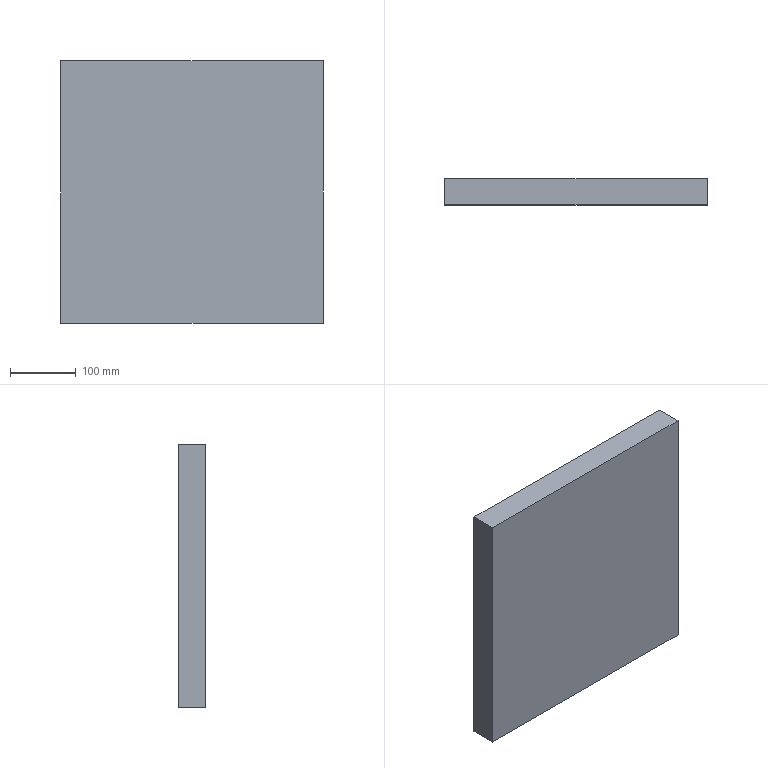Component | SolidWorks | DieBasePlate-1 | 1 solid | 6 faces | box 400 x 40 x 400 mm | volume 6400000 mm3 | plane 6
build123d program:
from build123d import *

# Parameters (mm, degrees)
SKETCH1_W           = 400
SKETCH1_H           = 400
BOSS_EXTRUDE1_DEPTH = 40


with BuildPart() as part:
    # Sketch1 → Boss-Extrude1 (new body)
    with BuildSketch(Plane.XY):
        with Locations((200, 200)):
            Rectangle(SKETCH1_W, SKETCH1_H)
    extrude(amount=BOSS_EXTRUDE1_DEPTH)


solid = part.part

# Placed as in the assembly
solid = solid.moved(Location((-377.951, 437.323, -195), (90, 0, 0)))
STEP:
#1=CARTESIAN_POINT('',(-14.88,15.643,-7.677));
#2=VERTEX_POINT('',#1);
#3=CARTESIAN_POINT('',(-14.88,15.643,8.071));
#4=VERTEX_POINT('',#3);
#5=CARTESIAN_POINT('',(-14.88,15.643,8.071));
#6=DIRECTION('',(0.,-0.,1.));
#7=VECTOR('',#6,39.37);
#8=LINE('',#5,#7);
#9=EDGE_CURVE('',#2,#4,#8,.T.);
#10=ORIENTED_EDGE('',*,*,#9,.T.);
#11=CARTESIAN_POINT('',(-14.88,17.217,8.071));
#12=VERTEX_POINT('',#11);
#13=CARTESIAN_POINT('',(-14.88,17.217,8.071));
#14=DIRECTION('',(-0.,-1.,-0.));
#15=VECTOR('',#14,39.37);
#16=LINE('',#13,#15);
#17=EDGE_CURVE('',#12,#4,#16,.T.);
#18=ORIENTED_EDGE('',*,*,#17,.F.);
#19=CARTESIAN_POINT('',(-14.88,17.217,-7.677));
#20=VERTEX_POINT('',#19);
#21=CARTESIAN_POINT('',(-14.88,17.217,8.071));
#22=DIRECTION('',(0.,-0.,1.));
#23=VECTOR('',#22,39.37);
#24=LINE('',#21,#23);
#25=EDGE_CURVE('',#20,#12,#24,.T.);
#26=ORIENTED_EDGE('',*,*,#25,.F.);
#27=CARTESIAN_POINT('',(-14.88,17.217,-7.677));
#28=DIRECTION('',(-0.,-1.,-0.));
#29=VECTOR('',#28,39.37);
#30=LINE('',#27,#29);
#31=EDGE_CURVE('',#20,#2,#30,.T.);
#32=ORIENTED_EDGE('',*,*,#31,.T.);
#33=EDGE_LOOP('',(#10,#18,#26,#32));
#34=FACE_OUTER_BOUND('',#33,.T.);
#35=CARTESIAN_POINT('',(-14.88,17.217,8.071));
#36=DIRECTION('',(1.,-0.,-0.));
#37=DIRECTION('',(-0.,-1.,-0.));
#38=AXIS2_PLACEMENT_3D('',#35,#36,#37);
#39=PLANE('',#38);
#40=ADVANCED_FACE('',(#34),#39,.F.);
#41=CARTESIAN_POINT('',(0.8681,15.643,8.071));
#42=VERTEX_POINT('',#41);
#43=CARTESIAN_POINT('',(-14.88,15.643,8.071));
#44=DIRECTION('',(1.,-0.,-0.));
#45=VECTOR('',#44,39.37);
#46=LINE('',#43,#45);
#47=EDGE_CURVE('',#4,#42,#46,.T.);
#48=ORIENTED_EDGE('',*,*,#47,.T.);
#49=CARTESIAN_POINT('',(0.8681,17.217,8.071));
#50=VERTEX_POINT('',#49);
#51=CARTESIAN_POINT('',(0.8681,17.217,8.071));
#52=DIRECTION('',(-0.,-1.,-0.));
#53=VECTOR('',#52,39.37);
#54=LINE('',#51,#53);
#55=EDGE_CURVE('',#50,#42,#54,.T.);
#56=ORIENTED_EDGE('',*,*,#55,.F.);
#57=CARTESIAN_POINT('',(-14.88,17.217,8.071));
#58=DIRECTION('',(1.,-0.,-0.));
#59=VECTOR('',#58,39.37);
#60=LINE('',#57,#59);
#61=EDGE_CURVE('',#12,#50,#60,.T.);
#62=ORIENTED_EDGE('',*,*,#61,.F.);
#63=ORIENTED_EDGE('',*,*,#17,.T.);
#64=EDGE_LOOP('',(#48,#56,#62,#63));
#65=FACE_OUTER_BOUND('',#64,.T.);
#66=CARTESIAN_POINT('',(-14.88,17.217,8.071));
#67=DIRECTION('',(-0.,0.,-1.));
#68=DIRECTION('',(0.,1.,0.));
#69=AXIS2_PLACEMENT_3D('',#66,#67,#68);
#70=PLANE('',#69);
#71=ADVANCED_FACE('',(#65),#70,.F.);
#72=CARTESIAN_POINT('',(0.8681,15.643,-7.677));
#73=VERTEX_POINT('',#72);
#74=CARTESIAN_POINT('',(0.8681,15.643,8.071));
#75=DIRECTION('',(-0.,0.,-1.));
#76=VECTOR('',#75,39.37);
#77=LINE('',#74,#76);
#78=EDGE_CURVE('',#42,#73,#77,.T.);
#79=ORIENTED_EDGE('',*,*,#78,.T.);
#80=CARTESIAN_POINT('',(0.8681,17.217,-7.677));
#81=VERTEX_POINT('',#80);
#82=CARTESIAN_POINT('',(0.8681,17.217,-7.677));
#83=DIRECTION('',(-0.,-1.,-0.));
#84=VECTOR('',#83,39.37);
#85=LINE('',#82,#84);
#86=EDGE_CURVE('',#81,#73,#85,.T.);
#87=ORIENTED_EDGE('',*,*,#86,.F.);
#88=CARTESIAN_POINT('',(0.8681,17.217,8.071));
#89=DIRECTION('',(-0.,0.,-1.));
#90=VECTOR('',#89,39.37);
#91=LINE('',#88,#90);
#92=EDGE_CURVE('',#50,#81,#91,.T.);
#93=ORIENTED_EDGE('',*,*,#92,.F.);
#94=ORIENTED_EDGE('',*,*,#55,.T.);
#95=EDGE_LOOP('',(#79,#87,#93,#94));
#96=FACE_OUTER_BOUND('',#95,.T.);
#97=CARTESIAN_POINT('',(0.8681,17.217,8.071));
#98=DIRECTION('',(-1.,0.,0.));
#99=DIRECTION('',(0.,1.,0.));
#100=AXIS2_PLACEMENT_3D('',#97,#98,#99);
#101=PLANE('',#100);
#102=ADVANCED_FACE('',(#96),#101,.F.);
#103=CARTESIAN_POINT('',(-14.88,15.643,-7.677));
#104=DIRECTION('',(-1.,0.,0.));
#105=VECTOR('',#104,39.37);
#106=LINE('',#103,#105);
#107=EDGE_CURVE('',#73,#2,#106,.T.);
#108=ORIENTED_EDGE('',*,*,#107,.T.);
#109=ORIENTED_EDGE('',*,*,#31,.F.);
#110=CARTESIAN_POINT('',(-14.88,17.217,-7.677));
#111=DIRECTION('',(-1.,0.,0.));
#112=VECTOR('',#111,39.37);
#113=LINE('',#110,#112);
#114=EDGE_CURVE('',#81,#20,#113,.T.);
#115=ORIENTED_EDGE('',*,*,#114,.F.);
#116=ORIENTED_EDGE('',*,*,#86,.T.);
#117=EDGE_LOOP('',(#108,#109,#115,#116));
#118=FACE_OUTER_BOUND('',#117,.T.);
#119=CARTESIAN_POINT('',(-14.88,17.217,-7.677));
#120=DIRECTION('',(0.,-0.,1.));
#121=DIRECTION('',(-0.,-1.,-0.));
#122=AXIS2_PLACEMENT_3D('',#119,#120,#121);
#123=PLANE('',#122);
#124=ADVANCED_FACE('',(#118),#123,.F.);
#125=ORIENTED_EDGE('',*,*,#25,.T.);
#126=ORIENTED_EDGE('',*,*,#61,.T.);
#127=ORIENTED_EDGE('',*,*,#92,.T.);
#128=ORIENTED_EDGE('',*,*,#114,.T.);
#129=EDGE_LOOP('',(#125,#126,#127,#128));
#130=FACE_OUTER_BOUND('',#129,.T.);
#131=CARTESIAN_POINT('',(-14.88,17.217,8.071));
#132=DIRECTION('',(-0.,-1.,-0.));
#133=DIRECTION('',(-1.,0.,0.));
#134=AXIS2_PLACEMENT_3D('',#131,#132,#133);
#135=PLANE('',#134);
#136=ADVANCED_FACE('',(#130),#135,.F.);
#137=ORIENTED_EDGE('',*,*,#9,.F.);
#138=ORIENTED_EDGE('',*,*,#107,.F.);
#139=ORIENTED_EDGE('',*,*,#78,.F.);
#140=ORIENTED_EDGE('',*,*,#47,.F.);
#141=EDGE_LOOP('',(#137,#138,#139,#140));
#142=FACE_OUTER_BOUND('',#141,.T.);
#143=CARTESIAN_POINT('',(-14.88,15.643,8.071));
#144=DIRECTION('',(-0.,-1.,-0.));
#145=DIRECTION('',(-1.,0.,0.));
#146=AXIS2_PLACEMENT_3D('',#143,#144,#145);
#147=PLANE('',#146);
#148=ADVANCED_FACE('',(#142),#147,.T.);
#149=CLOSED_SHELL('',(#40,#71,#102,#124,#136,#148));
#150=MANIFOLD_SOLID_BREP('',#149);
#151=CARTESIAN_POINT('',(0.,0.,0.));
#152=DIRECTION('',(0.,0.,1.));
#153=DIRECTION('',(1.,0.,0.));
#154=AXIS2_PLACEMENT_3D('',#151,#152,#153);
#155=(LENGTH_UNIT()NAMED_UNIT(*)SI_UNIT($,.METRE.));
#156=LENGTH_MEASURE_WITH_UNIT(LENGTH_MEASURE(0.0254),#155);
#157=DIMENSIONAL_EXPONENTS(1.,0.,0.,0.,0.,0.,0.);
#158=(CONVERSION_BASED_UNIT('',#156)LENGTH_UNIT()NAMED_UNIT(#157));
#159=UNCERTAINTY_MEASURE_WITH_UNIT(LENGTH_MEASURE(0.00001),#158,'','');
#160=(NAMED_UNIT(*)PLANE_ANGLE_UNIT()SI_UNIT($,.RADIAN.));
#161=(NAMED_UNIT(*)SI_UNIT($,.STERADIAN.)SOLID_ANGLE_UNIT());
#162=(GEOMETRIC_REPRESENTATION_CONTEXT(3)GLOBAL_UNCERTAINTY_ASSIGNED_CONTEXT((#159))GLOBAL_UNIT_ASSIGNED_CONTEXT((#158,#160,#161))REPRESENTATION_CONTEXT('',''));
#163=ADVANCED_BREP_SHAPE_REPRESENTATION('',(#150,#154),#162);
#164=COLOUR_RGB('',0.7922,0.8196,0.9333);
#165=FILL_AREA_STYLE_COLOUR('',#164);
#166=FILL_AREA_STYLE('',(#165));
#167=SURFACE_STYLE_FILL_AREA(#166);
#168=SURFACE_SIDE_STYLE('',(#167));
#169=SURFACE_STYLE_USAGE(.BOTH.,#168);
#170=PRESENTATION_STYLE_ASSIGNMENT((#169));
#171=STYLED_ITEM('',(#170),#150);
#172=(LENGTH_UNIT()NAMED_UNIT(*)SI_UNIT($,.METRE.));
#173=LENGTH_MEASURE_WITH_UNIT(LENGTH_MEASURE(0.0254),#172);
#174=DIMENSIONAL_EXPONENTS(1.,0.,0.,0.,0.,0.,0.);
#175=(CONVERSION_BASED_UNIT('',#173)LENGTH_UNIT()NAMED_UNIT(#174));
#176=UNCERTAINTY_MEASURE_WITH_UNIT(LENGTH_MEASURE(0.00001),#175,'','');
#177=(NAMED_UNIT(*)PLANE_ANGLE_UNIT()SI_UNIT($,.RADIAN.));
#178=(NAMED_UNIT(*)SI_UNIT($,.STERADIAN.)SOLID_ANGLE_UNIT());
#179=(GEOMETRIC_REPRESENTATION_CONTEXT(3)GLOBAL_UNCERTAINTY_ASSIGNED_CONTEXT((#176))GLOBAL_UNIT_ASSIGNED_CONTEXT((#175,#177,#178))REPRESENTATION_CONTEXT('',''));
#180=MECHANICAL_DESIGN_GEOMETRIC_PRESENTATION_REPRESENTATION('',(#171),#179);
#181=PRESENTATION_LAYER_ASSIGNMENT('','',(#171));